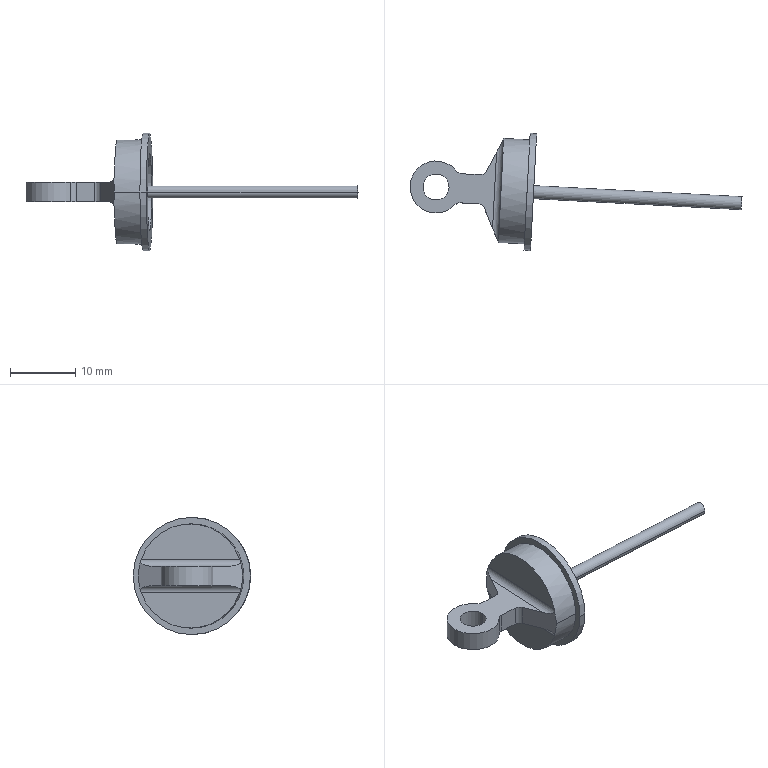Component | SolidWorks | WheelAssembly-1_DamperUpperEnd-1 | 1 solid | 29 faces | box 50.99 x 18.03 x 18 mm | volume 1080 mm3 | cylinder 17 | plane 12 | commonest cylinder face diameters 2 x8 16 x2 4 x2 18 x2 12 x2 8 x1
STEP:
#1=COLOUR_RGB('',0.7922,0.8196,0.9333);
#2=FILL_AREA_STYLE_COLOUR('',#1);
#3=FILL_AREA_STYLE('',(#2));
#4=SURFACE_STYLE_FILL_AREA(#3);
#5=SURFACE_SIDE_STYLE('',(#4));
#6=SURFACE_STYLE_USAGE(.BOTH.,#5);
#7=PRESENTATION_STYLE_ASSIGNMENT((#6));
#8=CARTESIAN_POINT('',(-12.976,-4.793,-22.066));
#9=VERTEX_POINT('',#8);
#10=CARTESIAN_POINT('',(-13.01,-5.422,-22.066));
#11=VERTEX_POINT('',#10);
#12=CARTESIAN_POINT('',(-12.993,-5.108,-22.066));
#13=DIRECTION('',(0.9986,-0.05275,-0.));
#14=DIRECTION('',(0.05275,0.9986,0.));
#15=AXIS2_PLACEMENT_3D('',#12,#13,#14);
#16=CIRCLE('',#15,0.315);
#17=EDGE_CURVE('',#9,#11,#16,.T.);
#18=ORIENTED_EDGE('',*,*,#17,.F.);
#19=CARTESIAN_POINT('',(-13.134,-4.785,-22.066));
#20=VERTEX_POINT('',#19);
#21=CARTESIAN_POINT('',(-12.819,-4.802,-22.066));
#22=DIRECTION('',(-0.9986,0.05275,0.));
#23=VECTOR('',#22,39.37);
#24=LINE('',#21,#23);
#25=EDGE_CURVE('',#9,#20,#24,.T.);
#26=ORIENTED_EDGE('',*,*,#25,.T.);
#27=CARTESIAN_POINT('',(-13.139,-4.795,-21.986));
#28=VERTEX_POINT('',#27);
#29=CARTESIAN_POINT('',(-13.139,-4.795,-21.986));
#30=CARTESIAN_POINT('',(-13.135,-4.788,-22.012));
#31=CARTESIAN_POINT('',(-13.134,-4.785,-22.039));
#32=CARTESIAN_POINT('',(-13.134,-4.785,-22.066));
#33=(BOUNDED_CURVE()B_SPLINE_CURVE(3,(#29,#30,#31,#32),.UNSPECIFIED.,.F.,.F.)B_SPLINE_CURVE_WITH_KNOTS((4,4),(6.028,6.283),.UNSPECIFIED.)CURVE()GEOMETRIC_REPRESENTATION_ITEM()RATIONAL_B_SPLINE_CURVE((1.,0.9946,0.9946,1.))REPRESENTATION_ITEM(''));
#34=EDGE_CURVE('',#28,#20,#33,.T.);
#35=ORIENTED_EDGE('',*,*,#34,.F.);
#36=CARTESIAN_POINT('',(-13.134,-4.801,-21.967));
#37=VERTEX_POINT('',#36);
#38=CARTESIAN_POINT('',(-13.139,-4.795,-21.986));
#39=CARTESIAN_POINT('',(-13.136,-4.797,-21.98));
#40=CARTESIAN_POINT('',(-13.134,-4.799,-21.974));
#41=CARTESIAN_POINT('',(-13.134,-4.801,-21.967));
#42=B_SPLINE_CURVE_WITH_KNOTS('',3,(#38,#39,#40,#41),.UNSPECIFIED.,.F.,.F.,(4,4),(0.,0.0005135),.UNSPECIFIED.);
#43=EDGE_CURVE('',#28,#37,#42,.T.);
#44=ORIENTED_EDGE('',*,*,#43,.T.);
#45=CARTESIAN_POINT('',(-13.166,-5.398,-21.967));
#46=VERTEX_POINT('',#45);
#47=CARTESIAN_POINT('',(-13.15,-5.1,-22.066));
#48=DIRECTION('',(-0.9986,0.05275,0.));
#49=DIRECTION('',(-0.05275,-0.9986,0.));
#50=AXIS2_PLACEMENT_3D('',#47,#48,#49);
#51=CIRCLE('',#50,0.315);
#52=EDGE_CURVE('',#46,#37,#51,.T.);
#53=ORIENTED_EDGE('',*,*,#52,.F.);
#54=CARTESIAN_POINT('',(-13.171,-5.404,-21.986));
#55=VERTEX_POINT('',#54);
#56=CARTESIAN_POINT('',(-13.166,-5.398,-21.967));
#57=CARTESIAN_POINT('',(-13.166,-5.4,-21.974));
#58=CARTESIAN_POINT('',(-13.168,-5.402,-21.98));
#59=CARTESIAN_POINT('',(-13.171,-5.404,-21.986));
#60=B_SPLINE_CURVE_WITH_KNOTS('',3,(#56,#57,#58,#59),.UNSPECIFIED.,.F.,.F.,(4,4),(0.,0.0005136),.UNSPECIFIED.);
#61=EDGE_CURVE('',#46,#55,#60,.T.);
#62=ORIENTED_EDGE('',*,*,#61,.T.);
#63=CARTESIAN_POINT('',(-13.167,-5.414,-22.066));
#64=VERTEX_POINT('',#63);
#65=CARTESIAN_POINT('',(-13.167,-5.414,-22.066));
#66=CARTESIAN_POINT('',(-13.167,-5.414,-22.039));
#67=CARTESIAN_POINT('',(-13.168,-5.411,-22.012));
#68=CARTESIAN_POINT('',(-13.171,-5.404,-21.986));
#69=(BOUNDED_CURVE()B_SPLINE_CURVE(3,(#65,#66,#67,#68),.UNSPECIFIED.,.F.,.F.)B_SPLINE_CURVE_WITH_KNOTS((4,4),(-0.,0.2556),.UNSPECIFIED.)CURVE()GEOMETRIC_REPRESENTATION_ITEM()RATIONAL_B_SPLINE_CURVE((1.,0.9946,0.9946,1.))REPRESENTATION_ITEM(''));
#70=EDGE_CURVE('',#64,#55,#69,.T.);
#71=ORIENTED_EDGE('',*,*,#70,.F.);
#72=CARTESIAN_POINT('',(-12.852,-5.431,-22.066));
#73=DIRECTION('',(-0.9986,0.05275,0.));
#74=VECTOR('',#73,39.37);
#75=LINE('',#72,#74);
#76=EDGE_CURVE('',#11,#64,#75,.T.);
#77=ORIENTED_EDGE('',*,*,#76,.F.);
#78=EDGE_LOOP('',(#18,#26,#35,#44,#53,#62,#71,#77));
#79=FACE_OUTER_BOUND('',#78,.T.);
#80=CARTESIAN_POINT('',(-12.836,-5.116,-22.066));
#81=DIRECTION('',(-0.9986,0.05275,0.));
#82=DIRECTION('',(-0.05275,-0.9986,0.));
#83=AXIS2_PLACEMENT_3D('',#80,#81,#82);
#84=CYLINDRICAL_SURFACE('',#83,0.315);
#85=ADVANCED_FACE('',(#79),#84,.T.);
#86=CARTESIAN_POINT('',(-13.465,-5.083,-22.007));
#87=VERTEX_POINT('',#86);
#88=CARTESIAN_POINT('',(-13.622,-5.075,-22.007));
#89=VERTEX_POINT('',#88);
#90=CARTESIAN_POINT('',(-13.543,-5.079,-22.007));
#91=DIRECTION('',(0.,0.,1.));
#92=DIRECTION('',(-0.9986,0.05275,0.));
#93=AXIS2_PLACEMENT_3D('',#90,#91,#92);
#94=CIRCLE('',#93,0.07874);
#95=EDGE_CURVE('',#87,#89,#94,.T.);
#96=ORIENTED_EDGE('',*,*,#95,.T.);
#97=CARTESIAN_POINT('',(-13.622,-5.075,-22.125));
#98=VERTEX_POINT('',#97);
#99=CARTESIAN_POINT('',(-13.622,-5.075,-22.007));
#100=DIRECTION('',(-0.,-0.,-1.));
#101=VECTOR('',#100,39.37);
#102=LINE('',#99,#101);
#103=EDGE_CURVE('',#89,#98,#102,.T.);
#104=ORIENTED_EDGE('',*,*,#103,.T.);
#105=CARTESIAN_POINT('',(-13.465,-5.083,-22.125));
#106=VERTEX_POINT('',#105);
#107=CARTESIAN_POINT('',(-13.543,-5.079,-22.125));
#108=DIRECTION('',(0.,0.,1.));
#109=DIRECTION('',(-0.9986,0.05275,0.));
#110=AXIS2_PLACEMENT_3D('',#107,#108,#109);
#111=CIRCLE('',#110,0.07874);
#112=EDGE_CURVE('',#106,#98,#111,.T.);
#113=ORIENTED_EDGE('',*,*,#112,.F.);
#114=CARTESIAN_POINT('',(-13.465,-5.083,-22.007));
#115=DIRECTION('',(-0.,-0.,-1.));
#116=VECTOR('',#115,39.37);
#117=LINE('',#114,#116);
#118=EDGE_CURVE('',#87,#106,#117,.T.);
#119=ORIENTED_EDGE('',*,*,#118,.F.);
#120=EDGE_LOOP('',(#96,#104,#113,#119));
#121=FACE_OUTER_BOUND('',#120,.T.);
#122=CARTESIAN_POINT('',(-13.543,-5.079,-22.007));
#123=DIRECTION('',(-0.,-0.,-1.));
#124=DIRECTION('',(0.9986,-0.05275,0.));
#125=AXIS2_PLACEMENT_3D('',#122,#123,#124);
#126=CYLINDRICAL_SURFACE('',#125,0.07874);
#127=ADVANCED_FACE('',(#121),#126,.F.);
#128=CARTESIAN_POINT('',(-12.974,-4.754,-22.066));
#129=VERTEX_POINT('',#128);
#130=CARTESIAN_POINT('',(-13.012,-5.462,-22.066));
#131=VERTEX_POINT('',#130);
#132=CARTESIAN_POINT('',(-12.993,-5.108,-22.066));
#133=DIRECTION('',(0.9986,-0.05275,-0.));
#134=DIRECTION('',(0.05275,0.9986,0.));
#135=AXIS2_PLACEMENT_3D('',#132,#133,#134);
#136=CIRCLE('',#135,0.3543);
#137=EDGE_CURVE('',#129,#131,#136,.T.);
#138=ORIENTED_EDGE('',*,*,#137,.T.);
#139=CARTESIAN_POINT('',(-12.972,-5.464,-22.066));
#140=VERTEX_POINT('',#139);
#141=CARTESIAN_POINT('',(-13.012,-5.462,-22.066));
#142=DIRECTION('',(0.9986,-0.05275,-0.));
#143=VECTOR('',#142,39.37);
#144=LINE('',#141,#143);
#145=EDGE_CURVE('',#131,#140,#144,.T.);
#146=ORIENTED_EDGE('',*,*,#145,.T.);
#147=CARTESIAN_POINT('',(-12.935,-4.756,-22.066));
#148=VERTEX_POINT('',#147);
#149=CARTESIAN_POINT('',(-12.954,-5.11,-22.066));
#150=DIRECTION('',(0.9986,-0.05275,-0.));
#151=DIRECTION('',(0.05275,0.9986,0.));
#152=AXIS2_PLACEMENT_3D('',#149,#150,#151);
#153=CIRCLE('',#152,0.3543);
#154=EDGE_CURVE('',#148,#140,#153,.T.);
#155=ORIENTED_EDGE('',*,*,#154,.F.);
#156=CARTESIAN_POINT('',(-12.974,-4.754,-22.066));
#157=DIRECTION('',(0.9986,-0.05275,-0.));
#158=VECTOR('',#157,39.37);
#159=LINE('',#156,#158);
#160=EDGE_CURVE('',#129,#148,#159,.T.);
#161=ORIENTED_EDGE('',*,*,#160,.F.);
#162=EDGE_LOOP('',(#138,#146,#155,#161));
#163=FACE_OUTER_BOUND('',#162,.T.);
#164=CARTESIAN_POINT('',(-12.993,-5.108,-22.066));
#165=DIRECTION('',(0.9986,-0.05275,-0.));
#166=DIRECTION('',(0.05275,0.9986,0.));
#167=AXIS2_PLACEMENT_3D('',#164,#165,#166);
#168=CYLINDRICAL_SURFACE('',#167,0.3543);
#169=ADVANCED_FACE('',(#163),#168,.T.);
#170=CARTESIAN_POINT('',(-11.693,-5.137,-22.066));
#171=VERTEX_POINT('',#170);
#172=CARTESIAN_POINT('',(-11.698,-5.216,-22.066));
#173=VERTEX_POINT('',#172);
#174=CARTESIAN_POINT('',(-11.695,-5.176,-22.066));
#175=DIRECTION('',(0.9986,-0.05275,-0.));
#176=DIRECTION('',(0.05275,0.9986,0.));
#177=AXIS2_PLACEMENT_3D('',#174,#175,#176);
#178=CIRCLE('',#177,0.03937);
#179=EDGE_CURVE('',#171,#173,#178,.T.);
#180=ORIENTED_EDGE('',*,*,#179,.F.);
#181=CARTESIAN_POINT('',(-13.069,-5.064,-22.066));
#182=VERTEX_POINT('',#181);
#183=CARTESIAN_POINT('',(-11.693,-5.137,-22.066));
#184=DIRECTION('',(-0.9986,0.05275,0.));
#185=VECTOR('',#184,39.37);
#186=LINE('',#183,#185);
#187=EDGE_CURVE('',#171,#182,#186,.T.);
#188=ORIENTED_EDGE('',*,*,#187,.T.);
#189=CARTESIAN_POINT('',(-13.074,-5.143,-22.066));
#190=VERTEX_POINT('',#189);
#191=CARTESIAN_POINT('',(-13.072,-5.104,-22.066));
#192=DIRECTION('',(0.9986,-0.05275,-0.));
#193=DIRECTION('',(-0.05275,-0.9986,0.));
#194=AXIS2_PLACEMENT_3D('',#191,#192,#193);
#195=CIRCLE('',#194,0.03937);
#196=EDGE_CURVE('',#182,#190,#195,.T.);
#197=ORIENTED_EDGE('',*,*,#196,.T.);
#198=CARTESIAN_POINT('',(-11.698,-5.216,-22.066));
#199=DIRECTION('',(-0.9986,0.05275,0.));
#200=VECTOR('',#199,39.37);
#201=LINE('',#198,#200);
#202=EDGE_CURVE('',#173,#190,#201,.T.);
#203=ORIENTED_EDGE('',*,*,#202,.F.);
#204=EDGE_LOOP('',(#180,#188,#197,#203));
#205=FACE_OUTER_BOUND('',#204,.T.);
#206=CARTESIAN_POINT('',(-11.695,-5.176,-22.066));
#207=DIRECTION('',(-0.9986,0.05275,0.));
#208=DIRECTION('',(-0.05275,-0.9986,0.));
#209=AXIS2_PLACEMENT_3D('',#206,#207,#208);
#210=CYLINDRICAL_SURFACE('',#209,0.03937);
#211=ADVANCED_FACE('',(#205),#210,.T.);
#212=CARTESIAN_POINT('',(-12.941,-4.874,-22.066));
#213=VERTEX_POINT('',#212);
#214=CARTESIAN_POINT('',(-12.966,-5.346,-22.066));
#215=VERTEX_POINT('',#214);
#216=CARTESIAN_POINT('',(-12.954,-5.11,-22.066));
#217=DIRECTION('',(-0.9986,0.05275,0.));
#218=DIRECTION('',(-0.05275,-0.9986,0.));
#219=AXIS2_PLACEMENT_3D('',#216,#217,#218);
#220=CIRCLE('',#219,0.2362);
#221=EDGE_CURVE('',#213,#215,#220,.T.);
#222=ORIENTED_EDGE('',*,*,#221,.F.);
#223=CARTESIAN_POINT('',(-13.059,-4.868,-22.066));
#224=VERTEX_POINT('',#223);
#225=CARTESIAN_POINT('',(-12.823,-4.88,-22.066));
#226=DIRECTION('',(-0.9986,0.05275,0.));
#227=VECTOR('',#226,39.37);
#228=LINE('',#225,#227);
#229=EDGE_CURVE('',#213,#224,#228,.T.);
#230=ORIENTED_EDGE('',*,*,#229,.T.);
#231=CARTESIAN_POINT('',(-13.084,-5.34,-22.066));
#232=VERTEX_POINT('',#231);
#233=CARTESIAN_POINT('',(-13.072,-5.104,-22.066));
#234=DIRECTION('',(-0.9986,0.05275,0.));
#235=DIRECTION('',(-0.05275,-0.9986,0.));
#236=AXIS2_PLACEMENT_3D('',#233,#234,#235);
#237=CIRCLE('',#236,0.2362);
#238=EDGE_CURVE('',#224,#232,#237,.T.);
#239=ORIENTED_EDGE('',*,*,#238,.T.);
#240=CARTESIAN_POINT('',(-12.848,-5.352,-22.066));
#241=DIRECTION('',(-0.9986,0.05275,0.));
#242=VECTOR('',#241,39.37);
#243=LINE('',#240,#242);
#244=EDGE_CURVE('',#215,#232,#243,.T.);
#245=ORIENTED_EDGE('',*,*,#244,.F.);
#246=EDGE_LOOP('',(#222,#230,#239,#245));
#247=FACE_OUTER_BOUND('',#246,.T.);
#248=CARTESIAN_POINT('',(-12.836,-5.116,-22.066));
#249=DIRECTION('',(-0.9986,0.05275,0.));
#250=DIRECTION('',(-0.05275,-0.9986,0.));
#251=AXIS2_PLACEMENT_3D('',#248,#249,#250);
#252=CYLINDRICAL_SURFACE('',#251,0.2362);
#253=ADVANCED_FACE('',(#247),#252,.F.);
#254=CARTESIAN_POINT('',(-12.954,-5.11,-22.066));
#255=DIRECTION('',(-0.9986,0.05275,0.));
#256=DIRECTION('',(-0.05275,-0.9986,0.));
#257=AXIS2_PLACEMENT_3D('',#254,#255,#256);
#258=CIRCLE('',#257,0.2362);
#259=EDGE_CURVE('',#215,#213,#258,.T.);
#260=ORIENTED_EDGE('',*,*,#259,.T.);
#261=ORIENTED_EDGE('',*,*,#221,.T.);
#262=EDGE_LOOP('',(#260,#261));
#263=FACE_BOUND('',#262,.T.);
#264=ORIENTED_EDGE('',*,*,#154,.T.);
#265=CARTESIAN_POINT('',(-12.954,-5.11,-22.066));
#266=DIRECTION('',(0.9986,-0.05275,-0.));
#267=DIRECTION('',(0.05275,0.9986,0.));
#268=AXIS2_PLACEMENT_3D('',#265,#266,#267);
#269=CIRCLE('',#268,0.3543);
#270=EDGE_CURVE('',#140,#148,#269,.T.);
#271=ORIENTED_EDGE('',*,*,#270,.T.);
#272=EDGE_LOOP('',(#264,#271));
#273=FACE_OUTER_BOUND('',#272,.T.);
#274=CARTESIAN_POINT('',(-12.954,-5.11,-22.066));
#275=DIRECTION('',(-0.9986,0.05275,0.));
#276=DIRECTION('',(-0.05275,-0.9986,0.));
#277=AXIS2_PLACEMENT_3D('',#274,#275,#276);
#278=PLANE('',#277);
#279=ADVANCED_FACE('',(#263,#273),#278,.F.);
#280=ORIENTED_EDGE('',*,*,#229,.F.);
#281=ORIENTED_EDGE('',*,*,#259,.F.);
#282=ORIENTED_EDGE('',*,*,#244,.T.);
#283=CARTESIAN_POINT('',(-13.072,-5.104,-22.066));
#284=DIRECTION('',(-0.9986,0.05275,0.));
#285=DIRECTION('',(-0.05275,-0.9986,0.));
#286=AXIS2_PLACEMENT_3D('',#283,#284,#285);
#287=CIRCLE('',#286,0.2362);
#288=EDGE_CURVE('',#232,#224,#287,.T.);
#289=ORIENTED_EDGE('',*,*,#288,.T.);
#290=EDGE_LOOP('',(#280,#281,#282,#289));
#291=FACE_OUTER_BOUND('',#290,.T.);
#292=CARTESIAN_POINT('',(-12.836,-5.116,-22.066));
#293=DIRECTION('',(-0.9986,0.05275,0.));
#294=DIRECTION('',(-0.05275,-0.9986,0.));
#295=AXIS2_PLACEMENT_3D('',#292,#293,#294);
#296=CYLINDRICAL_SURFACE('',#295,0.2362);
#297=ADVANCED_FACE('',(#291),#296,.F.);
#298=CARTESIAN_POINT('',(-13.072,-5.104,-22.066));
#299=DIRECTION('',(0.9986,-0.05275,-0.));
#300=DIRECTION('',(-0.05275,-0.9986,0.));
#301=AXIS2_PLACEMENT_3D('',#298,#299,#300);
#302=CIRCLE('',#301,0.03937);
#303=EDGE_CURVE('',#190,#182,#302,.T.);
#304=ORIENTED_EDGE('',*,*,#303,.F.);
#305=ORIENTED_EDGE('',*,*,#196,.F.);
#306=EDGE_LOOP('',(#304,#305));
#307=FACE_BOUND('',#306,.T.);
#308=ORIENTED_EDGE('',*,*,#288,.F.);
#309=ORIENTED_EDGE('',*,*,#238,.F.);
#310=EDGE_LOOP('',(#308,#309));
#311=FACE_OUTER_BOUND('',#310,.T.);
#312=CARTESIAN_POINT('',(-13.072,-5.104,-22.066));
#313=DIRECTION('',(-0.9986,0.05275,0.));
#314=DIRECTION('',(-0.05275,-0.9986,0.));
#315=AXIS2_PLACEMENT_3D('',#312,#313,#314);
#316=PLANE('',#315);
#317=ADVANCED_FACE('',(#307,#311),#316,.F.);
#318=ORIENTED_EDGE('',*,*,#187,.F.);
#319=CARTESIAN_POINT('',(-11.695,-5.176,-22.066));
#320=DIRECTION('',(0.9986,-0.05275,-0.));
#321=DIRECTION('',(0.05275,0.9986,0.));
#322=AXIS2_PLACEMENT_3D('',#319,#320,#321);
#323=CIRCLE('',#322,0.03937);
#324=EDGE_CURVE('',#173,#171,#323,.T.);
#325=ORIENTED_EDGE('',*,*,#324,.F.);
#326=ORIENTED_EDGE('',*,*,#202,.T.);
#327=ORIENTED_EDGE('',*,*,#303,.T.);
#328=EDGE_LOOP('',(#318,#325,#326,#327));
#329=FACE_OUTER_BOUND('',#328,.T.);
#330=CARTESIAN_POINT('',(-11.695,-5.176,-22.066));
#331=DIRECTION('',(-0.9986,0.05275,0.));
#332=DIRECTION('',(-0.05275,-0.9986,0.));
#333=AXIS2_PLACEMENT_3D('',#330,#331,#332);
#334=CYLINDRICAL_SURFACE('',#333,0.03937);
#335=ADVANCED_FACE('',(#329),#334,.T.);
#336=ORIENTED_EDGE('',*,*,#324,.T.);
#337=ORIENTED_EDGE('',*,*,#179,.T.);
#338=EDGE_LOOP('',(#336,#337));
#339=FACE_OUTER_BOUND('',#338,.T.);
#340=CARTESIAN_POINT('',(-11.695,-5.176,-22.066));
#341=DIRECTION('',(0.9986,-0.05275,-0.));
#342=DIRECTION('',(0.05275,0.9986,-0.));
#343=AXIS2_PLACEMENT_3D('',#340,#341,#342);
#344=PLANE('',#343);
#345=ADVANCED_FACE('',(#339),#344,.T.);
#346=ORIENTED_EDGE('',*,*,#145,.F.);
#347=CARTESIAN_POINT('',(-12.993,-5.108,-22.066));
#348=DIRECTION('',(0.9986,-0.05275,-0.));
#349=DIRECTION('',(0.05275,0.9986,0.));
#350=AXIS2_PLACEMENT_3D('',#347,#348,#349);
#351=CIRCLE('',#350,0.3543);
#352=EDGE_CURVE('',#131,#129,#351,.T.);
#353=ORIENTED_EDGE('',*,*,#352,.T.);
#354=ORIENTED_EDGE('',*,*,#160,.T.);
#355=ORIENTED_EDGE('',*,*,#270,.F.);
#356=EDGE_LOOP('',(#346,#353,#354,#355));
#357=FACE_OUTER_BOUND('',#356,.T.);
#358=CARTESIAN_POINT('',(-12.993,-5.108,-22.066));
#359=DIRECTION('',(0.9986,-0.05275,-0.));
#360=DIRECTION('',(0.05275,0.9986,0.));
#361=AXIS2_PLACEMENT_3D('',#358,#359,#360);
#362=CYLINDRICAL_SURFACE('',#361,0.3543);
#363=ADVANCED_FACE('',(#357),#362,.T.);
#364=CARTESIAN_POINT('',(-12.993,-5.108,-22.066));
#365=DIRECTION('',(0.9986,-0.05275,-0.));
#366=DIRECTION('',(0.05275,0.9986,0.));
#367=AXIS2_PLACEMENT_3D('',#364,#365,#366);
#368=CIRCLE('',#367,0.315);
#369=EDGE_CURVE('',#11,#9,#368,.T.);
#370=ORIENTED_EDGE('',*,*,#369,.T.);
#371=ORIENTED_EDGE('',*,*,#17,.T.);
#372=EDGE_LOOP('',(#370,#371));
#373=FACE_BOUND('',#372,.T.);
#374=ORIENTED_EDGE('',*,*,#137,.F.);
#375=ORIENTED_EDGE('',*,*,#352,.F.);
#376=EDGE_LOOP('',(#374,#375));
#377=FACE_OUTER_BOUND('',#376,.T.);
#378=CARTESIAN_POINT('',(-12.993,-5.108,-22.066));
#379=DIRECTION('',(0.9986,-0.05275,-0.));
#380=DIRECTION('',(0.05275,0.9986,-0.));
#381=AXIS2_PLACEMENT_3D('',#378,#379,#380);
#382=PLANE('',#381);
#383=ADVANCED_FACE('',(#373,#377),#382,.F.);
#384=ORIENTED_EDGE('',*,*,#103,.F.);
#385=CARTESIAN_POINT('',(-13.543,-5.079,-22.007));
#386=DIRECTION('',(0.,0.,1.));
#387=DIRECTION('',(-0.9986,0.05275,0.));
#388=AXIS2_PLACEMENT_3D('',#385,#386,#387);
#389=CIRCLE('',#388,0.07874);
#390=EDGE_CURVE('',#89,#87,#389,.T.);
#391=ORIENTED_EDGE('',*,*,#390,.T.);
#392=ORIENTED_EDGE('',*,*,#118,.T.);
#393=CARTESIAN_POINT('',(-13.543,-5.079,-22.125));
#394=DIRECTION('',(0.,0.,1.));
#395=DIRECTION('',(-0.9986,0.05275,0.));
#396=AXIS2_PLACEMENT_3D('',#393,#394,#395);
#397=CIRCLE('',#396,0.07874);
#398=EDGE_CURVE('',#98,#106,#397,.T.);
#399=ORIENTED_EDGE('',*,*,#398,.F.);
#400=EDGE_LOOP('',(#384,#391,#392,#399));
#401=FACE_OUTER_BOUND('',#400,.T.);
#402=CARTESIAN_POINT('',(-13.543,-5.079,-22.007));
#403=DIRECTION('',(-0.,-0.,-1.));
#404=DIRECTION('',(0.9986,-0.05275,0.));
#405=AXIS2_PLACEMENT_3D('',#402,#403,#404);
#406=CYLINDRICAL_SURFACE('',#405,0.07874);
#407=ADVANCED_FACE('',(#401),#406,.F.);
#408=CARTESIAN_POINT('',(-13.398,-5.175,-22.007));
#409=VERTEX_POINT('',#408);
#410=CARTESIAN_POINT('',(-13.285,-5.181,-22.007));
#411=VERTEX_POINT('',#410);
#412=CARTESIAN_POINT('',(-13.26,-5.182,-22.007));
#413=DIRECTION('',(0.9986,-0.05275,-0.));
#414=VECTOR('',#413,39.37);
#415=LINE('',#412,#414);
#416=EDGE_CURVE('',#409,#411,#415,.T.);
#417=ORIENTED_EDGE('',*,*,#416,.F.);
#418=CARTESIAN_POINT('',(-13.398,-5.175,-22.125));
#419=VERTEX_POINT('',#418);
#420=CARTESIAN_POINT('',(-13.398,-5.175,-22.125));
#421=DIRECTION('',(-0.,-0.,-1.));
#422=VECTOR('',#421,39.37);
#423=LINE('',#420,#422);
#424=EDGE_CURVE('',#409,#419,#423,.T.);
#425=ORIENTED_EDGE('',*,*,#424,.T.);
#426=CARTESIAN_POINT('',(-13.285,-5.181,-22.125));
#427=VERTEX_POINT('',#426);
#428=CARTESIAN_POINT('',(-13.26,-5.182,-22.125));
#429=DIRECTION('',(0.9986,-0.05275,-0.));
#430=VECTOR('',#429,39.37);
#431=LINE('',#428,#430);
#432=EDGE_CURVE('',#419,#427,#431,.T.);
#433=ORIENTED_EDGE('',*,*,#432,.T.);
#434=CARTESIAN_POINT('',(-13.285,-5.181,-22.007));
#435=DIRECTION('',(0.,0.,1.));
#436=VECTOR('',#435,39.37);
#437=LINE('',#434,#436);
#438=EDGE_CURVE('',#427,#411,#437,.T.);
#439=ORIENTED_EDGE('',*,*,#438,.T.);
#440=EDGE_LOOP('',(#417,#425,#433,#439));
#441=FACE_OUTER_BOUND('',#440,.T.);
#442=CARTESIAN_POINT('',(-13.26,-5.182,-22.007));
#443=DIRECTION('',(0.05275,0.9986,-0.));
#444=DIRECTION('',(-0.9986,0.05275,0.));
#445=AXIS2_PLACEMENT_3D('',#442,#443,#444);
#446=PLANE('',#445);
#447=ADVANCED_FACE('',(#441),#446,.F.);
#448=CARTESIAN_POINT('',(-13.429,-5.187,-22.007));
#449=VERTEX_POINT('',#448);
#450=CARTESIAN_POINT('',(-13.4,-5.214,-22.007));
#451=DIRECTION('',(-0.,-0.,-1.));
#452=DIRECTION('',(-0.9986,0.05275,0.));
#453=AXIS2_PLACEMENT_3D('',#450,#451,#452);
#454=CIRCLE('',#453,0.03937);
#455=EDGE_CURVE('',#449,#409,#454,.T.);
#456=ORIENTED_EDGE('',*,*,#455,.F.);
#457=CARTESIAN_POINT('',(-13.429,-5.187,-22.125));
#458=VERTEX_POINT('',#457);
#459=CARTESIAN_POINT('',(-13.429,-5.187,-22.007));
#460=DIRECTION('',(0.,0.,1.));
#461=VECTOR('',#460,39.37);
#462=LINE('',#459,#461);
#463=EDGE_CURVE('',#458,#449,#462,.T.);
#464=ORIENTED_EDGE('',*,*,#463,.F.);
#465=CARTESIAN_POINT('',(-13.4,-5.214,-22.125));
#466=DIRECTION('',(0.,0.,1.));
#467=DIRECTION('',(-0.9986,0.05275,0.));
#468=AXIS2_PLACEMENT_3D('',#465,#466,#467);
#469=CIRCLE('',#468,0.03937);
#470=EDGE_CURVE('',#419,#458,#469,.T.);
#471=ORIENTED_EDGE('',*,*,#470,.F.);
#472=ORIENTED_EDGE('',*,*,#424,.F.);
#473=EDGE_LOOP('',(#456,#464,#471,#472));
#474=FACE_OUTER_BOUND('',#473,.T.);
#475=CARTESIAN_POINT('',(-13.4,-5.214,-22.007));
#476=DIRECTION('',(-0.,-0.,-1.));
#477=DIRECTION('',(0.9986,-0.05275,0.));
#478=AXIS2_PLACEMENT_3D('',#475,#476,#477);
#479=CYLINDRICAL_SURFACE('',#478,0.03937);
#480=ADVANCED_FACE('',(#474),#479,.F.);
#481=CARTESIAN_POINT('',(-13.418,-4.983,-22.007));
#482=VERTEX_POINT('',#481);
#483=CARTESIAN_POINT('',(-13.543,-5.079,-22.007));
#484=DIRECTION('',(0.,0.,1.));
#485=DIRECTION('',(-0.9986,0.05275,0.));
#486=AXIS2_PLACEMENT_3D('',#483,#484,#485);
#487=CIRCLE('',#486,0.1575);
#488=EDGE_CURVE('',#482,#449,#487,.T.);
#489=ORIENTED_EDGE('',*,*,#488,.F.);
#490=CARTESIAN_POINT('',(-13.418,-4.983,-22.125));
#491=VERTEX_POINT('',#490);
#492=CARTESIAN_POINT('',(-13.418,-4.983,-22.007));
#493=DIRECTION('',(-0.,-0.,-1.));
#494=VECTOR('',#493,39.37);
#495=LINE('',#492,#494);
#496=EDGE_CURVE('',#482,#491,#495,.T.);
#497=ORIENTED_EDGE('',*,*,#496,.T.);
#498=CARTESIAN_POINT('',(-13.543,-5.079,-22.125));
#499=DIRECTION('',(0.,0.,1.));
#500=DIRECTION('',(-0.9986,0.05275,0.));
#501=AXIS2_PLACEMENT_3D('',#498,#499,#500);
#502=CIRCLE('',#501,0.1575);
#503=EDGE_CURVE('',#491,#458,#502,.T.);
#504=ORIENTED_EDGE('',*,*,#503,.T.);
#505=ORIENTED_EDGE('',*,*,#463,.T.);
#506=EDGE_LOOP('',(#489,#497,#504,#505));
#507=FACE_OUTER_BOUND('',#506,.T.);
#508=CARTESIAN_POINT('',(-13.543,-5.079,-22.007));
#509=DIRECTION('',(-0.,-0.,-1.));
#510=DIRECTION('',(0.9986,-0.05275,0.));
#511=AXIS2_PLACEMENT_3D('',#508,#509,#510);
#512=CYLINDRICAL_SURFACE('',#511,0.1575);
#513=ADVANCED_FACE('',(#507),#512,.T.);
#514=CARTESIAN_POINT('',(-13.389,-4.999,-22.007));
#515=VERTEX_POINT('',#514);
#516=CARTESIAN_POINT('',(-13.387,-4.959,-22.007));
#517=DIRECTION('',(-0.,-0.,-1.));
#518=DIRECTION('',(-0.9986,0.05275,0.));
#519=AXIS2_PLACEMENT_3D('',#516,#517,#518);
#520=CIRCLE('',#519,0.03937);
#521=EDGE_CURVE('',#515,#482,#520,.T.);
#522=ORIENTED_EDGE('',*,*,#521,.F.);
#523=CARTESIAN_POINT('',(-13.389,-4.999,-22.125));
#524=VERTEX_POINT('',#523);
#525=CARTESIAN_POINT('',(-13.389,-4.999,-22.007));
#526=DIRECTION('',(0.,0.,1.));
#527=VECTOR('',#526,39.37);
#528=LINE('',#525,#527);
#529=EDGE_CURVE('',#524,#515,#528,.T.);
#530=ORIENTED_EDGE('',*,*,#529,.F.);
#531=CARTESIAN_POINT('',(-13.387,-4.959,-22.125));
#532=DIRECTION('',(0.,0.,1.));
#533=DIRECTION('',(-0.9986,0.05275,0.));
#534=AXIS2_PLACEMENT_3D('',#531,#532,#533);
#535=CIRCLE('',#534,0.03937);
#536=EDGE_CURVE('',#491,#524,#535,.T.);
#537=ORIENTED_EDGE('',*,*,#536,.F.);
#538=ORIENTED_EDGE('',*,*,#496,.F.);
#539=EDGE_LOOP('',(#522,#530,#537,#538));
#540=FACE_OUTER_BOUND('',#539,.T.);
#541=CARTESIAN_POINT('',(-13.387,-4.959,-22.007));
#542=DIRECTION('',(-0.,-0.,-1.));
#543=DIRECTION('',(0.9986,-0.05275,0.));
#544=AXIS2_PLACEMENT_3D('',#541,#542,#543);
#545=CYLINDRICAL_SURFACE('',#544,0.03937);
#546=ADVANCED_FACE('',(#540),#545,.F.);
#547=CARTESIAN_POINT('',(-13.276,-5.005,-22.007));
#548=VERTEX_POINT('',#547);
#549=CARTESIAN_POINT('',(-13.251,-5.006,-22.007));
#550=DIRECTION('',(-0.9986,0.05275,0.));
#551=VECTOR('',#550,39.37);
#552=LINE('',#549,#551);
#553=EDGE_CURVE('',#548,#515,#552,.T.);
#554=ORIENTED_EDGE('',*,*,#553,.F.);
#555=CARTESIAN_POINT('',(-13.276,-5.005,-22.125));
#556=VERTEX_POINT('',#555);
#557=CARTESIAN_POINT('',(-13.276,-5.005,-22.125));
#558=DIRECTION('',(-0.,-0.,-1.));
#559=VECTOR('',#558,39.37);
#560=LINE('',#557,#559);
#561=EDGE_CURVE('',#548,#556,#560,.T.);
#562=ORIENTED_EDGE('',*,*,#561,.T.);
#563=CARTESIAN_POINT('',(-13.251,-5.006,-22.125));
#564=DIRECTION('',(-0.9986,0.05275,0.));
#565=VECTOR('',#564,39.37);
#566=LINE('',#563,#565);
#567=EDGE_CURVE('',#556,#524,#566,.T.);
#568=ORIENTED_EDGE('',*,*,#567,.T.);
#569=ORIENTED_EDGE('',*,*,#529,.T.);
#570=EDGE_LOOP('',(#554,#562,#568,#569));
#571=FACE_OUTER_BOUND('',#570,.T.);
#572=CARTESIAN_POINT('',(-13.251,-5.006,-22.007));
#573=DIRECTION('',(-0.05275,-0.9986,0.));
#574=DIRECTION('',(0.9986,-0.05275,-0.));
#575=AXIS2_PLACEMENT_3D('',#572,#573,#574);
#576=PLANE('',#575);
#577=ADVANCED_FACE('',(#571),#576,.F.);
#578=CARTESIAN_POINT('',(-13.239,-4.984,-22.007));
#579=VERTEX_POINT('',#578);
#580=CARTESIAN_POINT('',(-13.274,-4.965,-22.007));
#581=DIRECTION('',(-0.,-0.,-1.));
#582=DIRECTION('',(-0.9986,0.05275,0.));
#583=AXIS2_PLACEMENT_3D('',#580,#581,#582);
#584=CIRCLE('',#583,0.03937);
#585=EDGE_CURVE('',#579,#548,#584,.T.);
#586=ORIENTED_EDGE('',*,*,#585,.F.);
#587=CARTESIAN_POINT('',(-13.239,-4.984,-22.125));
#588=VERTEX_POINT('',#587);
#589=CARTESIAN_POINT('',(-13.239,-4.984,-22.007));
#590=DIRECTION('',(0.,0.,1.));
#591=VECTOR('',#590,39.37);
#592=LINE('',#589,#591);
#593=EDGE_CURVE('',#588,#579,#592,.T.);
#594=ORIENTED_EDGE('',*,*,#593,.F.);
#595=CARTESIAN_POINT('',(-13.274,-4.965,-22.125));
#596=DIRECTION('',(0.,0.,1.));
#597=DIRECTION('',(-0.9986,0.05275,0.));
#598=AXIS2_PLACEMENT_3D('',#595,#596,#597);
#599=CIRCLE('',#598,0.03937);
#600=EDGE_CURVE('',#556,#588,#599,.T.);
#601=ORIENTED_EDGE('',*,*,#600,.F.);
#602=ORIENTED_EDGE('',*,*,#561,.F.);
#603=EDGE_LOOP('',(#586,#594,#601,#602));
#604=FACE_OUTER_BOUND('',#603,.T.);
#605=CARTESIAN_POINT('',(-13.274,-4.965,-22.007));
#606=DIRECTION('',(0.,0.,1.));
#607=DIRECTION('',(-0.9986,0.05275,0.));
#608=AXIS2_PLACEMENT_3D('',#605,#606,#607);
#609=CYLINDRICAL_SURFACE('',#608,0.03937);
#610=ADVANCED_FACE('',(#604),#609,.F.);
#611=CARTESIAN_POINT('',(-13.177,-4.867,-22.125));
#612=VERTEX_POINT('',#611);
#613=CARTESIAN_POINT('',(-13.134,-4.785,-22.125));
#614=DIRECTION('',(-0.4698,-0.8828,0.));
#615=VECTOR('',#614,39.37);
#616=LINE('',#613,#615);
#617=EDGE_CURVE('',#612,#588,#616,.T.);
#618=ORIENTED_EDGE('',*,*,#617,.F.);
#619=CARTESIAN_POINT('',(-13.202,-5.328,-22.125));
#620=VERTEX_POINT('',#619);
#621=CARTESIAN_POINT('',(-13.189,-5.097,-22.125));
#622=DIRECTION('',(-0.05275,-0.9986,0.));
#623=VECTOR('',#622,39.37);
#624=LINE('',#621,#623);
#625=EDGE_CURVE('',#612,#620,#624,.T.);
#626=ORIENTED_EDGE('',*,*,#625,.T.);
#627=CARTESIAN_POINT('',(-13.251,-5.205,-22.125));
#628=VERTEX_POINT('',#627);
#629=CARTESIAN_POINT('',(-13.167,-5.414,-22.125));
#630=DIRECTION('',(0.3742,-0.9273,0.));
#631=VECTOR('',#630,39.37);
#632=LINE('',#629,#631);
#633=EDGE_CURVE('',#628,#620,#632,.T.);
#634=ORIENTED_EDGE('',*,*,#633,.F.);
#635=CARTESIAN_POINT('',(-13.288,-5.22,-22.125));
#636=DIRECTION('',(0.,0.,1.));
#637=DIRECTION('',(-0.9986,0.05275,0.));
#638=AXIS2_PLACEMENT_3D('',#635,#636,#637);
#639=CIRCLE('',#638,0.03937);
#640=EDGE_CURVE('',#628,#427,#639,.T.);
#641=ORIENTED_EDGE('',*,*,#640,.T.);
#642=ORIENTED_EDGE('',*,*,#432,.F.);
#643=ORIENTED_EDGE('',*,*,#470,.T.);
#644=ORIENTED_EDGE('',*,*,#503,.F.);
#645=ORIENTED_EDGE('',*,*,#536,.T.);
#646=ORIENTED_EDGE('',*,*,#567,.F.);
#647=ORIENTED_EDGE('',*,*,#600,.T.);
#648=EDGE_LOOP('',(#618,#626,#634,#641,#642,#643,#644,#645,#646,#647));
#649=FACE_OUTER_BOUND('',#648,.T.);
#650=ORIENTED_EDGE('',*,*,#112,.T.);
#651=ORIENTED_EDGE('',*,*,#398,.T.);
#652=EDGE_LOOP('',(#650,#651));
#653=FACE_BOUND('',#652,.T.);
#654=CARTESIAN_POINT('',(-13.543,-5.079,-22.125));
#655=DIRECTION('',(0.,0.,1.));
#656=DIRECTION('',(-0.9986,0.05275,0.));
#657=AXIS2_PLACEMENT_3D('',#654,#655,#656);
#658=PLANE('',#657);
#659=ADVANCED_FACE('',(#649,#653),#658,.F.);
#660=CARTESIAN_POINT('',(-13.251,-5.205,-22.007));
#661=VERTEX_POINT('',#660);
#662=CARTESIAN_POINT('',(-13.288,-5.22,-22.007));
#663=DIRECTION('',(-0.,-0.,-1.));
#664=DIRECTION('',(-0.9986,0.05275,0.));
#665=AXIS2_PLACEMENT_3D('',#662,#663,#664);
#666=CIRCLE('',#665,0.03937);
#667=EDGE_CURVE('',#411,#661,#666,.T.);
#668=ORIENTED_EDGE('',*,*,#667,.F.);
#669=ORIENTED_EDGE('',*,*,#438,.F.);
#670=ORIENTED_EDGE('',*,*,#640,.F.);
#671=CARTESIAN_POINT('',(-13.251,-5.205,-22.125));
#672=DIRECTION('',(-0.,-0.,-1.));
#673=VECTOR('',#672,39.37);
#674=LINE('',#671,#673);
#675=EDGE_CURVE('',#661,#628,#674,.T.);
#676=ORIENTED_EDGE('',*,*,#675,.F.);
#677=EDGE_LOOP('',(#668,#669,#670,#676));
#678=FACE_OUTER_BOUND('',#677,.T.);
#679=CARTESIAN_POINT('',(-13.288,-5.22,-22.007));
#680=DIRECTION('',(0.,0.,1.));
#681=DIRECTION('',(-0.9986,0.05275,0.));
#682=AXIS2_PLACEMENT_3D('',#679,#680,#681);
#683=CYLINDRICAL_SURFACE('',#682,0.03937);
#684=ADVANCED_FACE('',(#678),#683,.F.);
#685=CARTESIAN_POINT('',(-13.202,-5.328,-22.007));
#686=VERTEX_POINT('',#685);
#687=CARTESIAN_POINT('',(-13.167,-5.414,-22.007));
#688=DIRECTION('',(0.3742,-0.9273,0.));
#689=VECTOR('',#688,39.37);
#690=LINE('',#687,#689);
#691=EDGE_CURVE('',#661,#686,#690,.T.);
#692=ORIENTED_EDGE('',*,*,#691,.T.);
#693=CARTESIAN_POINT('',(-13.177,-4.867,-22.007));
#694=VERTEX_POINT('',#693);
#695=CARTESIAN_POINT('',(-13.173,-4.788,-22.007));
#696=DIRECTION('',(0.05275,0.9986,-0.));
#697=VECTOR('',#696,39.37);
#698=LINE('',#695,#697);
#699=EDGE_CURVE('',#686,#694,#698,.T.);
#700=ORIENTED_EDGE('',*,*,#699,.T.);
#701=CARTESIAN_POINT('',(-13.134,-4.785,-22.007));
#702=DIRECTION('',(-0.4698,-0.8828,0.));
#703=VECTOR('',#702,39.37);
#704=LINE('',#701,#703);
#705=EDGE_CURVE('',#694,#579,#704,.T.);
#706=ORIENTED_EDGE('',*,*,#705,.T.);
#707=ORIENTED_EDGE('',*,*,#585,.T.);
#708=ORIENTED_EDGE('',*,*,#553,.T.);
#709=ORIENTED_EDGE('',*,*,#521,.T.);
#710=ORIENTED_EDGE('',*,*,#488,.T.);
#711=ORIENTED_EDGE('',*,*,#455,.T.);
#712=ORIENTED_EDGE('',*,*,#416,.T.);
#713=ORIENTED_EDGE('',*,*,#667,.T.);
#714=EDGE_LOOP('',(#692,#700,#706,#707,#708,#709,#710,#711,#712,#713));
#715=FACE_OUTER_BOUND('',#714,.T.);
#716=ORIENTED_EDGE('',*,*,#95,.F.);
#717=ORIENTED_EDGE('',*,*,#390,.F.);
#718=EDGE_LOOP('',(#716,#717));
#719=FACE_BOUND('',#718,.T.);
#720=CARTESIAN_POINT('',(-13.543,-5.079,-22.007));
#721=DIRECTION('',(0.,0.,1.));
#722=DIRECTION('',(-0.9986,0.05275,0.));
#723=AXIS2_PLACEMENT_3D('',#720,#721,#722);
#724=PLANE('',#723);
#725=ADVANCED_FACE('',(#715,#719),#724,.T.);
#726=ORIENTED_EDGE('',*,*,#34,.T.);
#727=CARTESIAN_POINT('',(-13.139,-4.795,-22.145));
#728=VERTEX_POINT('',#727);
#729=CARTESIAN_POINT('',(-13.134,-4.785,-22.066));
#730=CARTESIAN_POINT('',(-13.134,-4.785,-22.093));
#731=CARTESIAN_POINT('',(-13.135,-4.788,-22.119));
#732=CARTESIAN_POINT('',(-13.139,-4.795,-22.145));
#733=(BOUNDED_CURVE()B_SPLINE_CURVE(3,(#729,#730,#731,#732),.UNSPECIFIED.,.F.,.F.)B_SPLINE_CURVE_WITH_KNOTS((4,4),(-0.,0.2556),.UNSPECIFIED.)CURVE()GEOMETRIC_REPRESENTATION_ITEM()RATIONAL_B_SPLINE_CURVE((1.,0.9946,0.9946,1.))REPRESENTATION_ITEM(''));
#734=EDGE_CURVE('',#20,#728,#733,.T.);
#735=ORIENTED_EDGE('',*,*,#734,.T.);
#736=CARTESIAN_POINT('',(-13.139,-4.795,-22.145));
#737=CARTESIAN_POINT('',(-13.147,-4.81,-22.132));
#738=CARTESIAN_POINT('',(-13.161,-4.836,-22.125));
#739=CARTESIAN_POINT('',(-13.177,-4.867,-22.125));
#740=(BOUNDED_CURVE()B_SPLINE_CURVE(3,(#736,#737,#738,#739),.UNSPECIFIED.,.F.,.F.)B_SPLINE_CURVE_WITH_KNOTS((4,4),(0.4975,1.571),.UNSPECIFIED.)CURVE()GEOMETRIC_REPRESENTATION_ITEM()RATIONAL_B_SPLINE_CURVE((1.,0.9063,0.9063,1.))REPRESENTATION_ITEM(''));
#741=EDGE_CURVE('',#728,#612,#740,.T.);
#742=ORIENTED_EDGE('',*,*,#741,.T.);
#743=ORIENTED_EDGE('',*,*,#617,.T.);
#744=ORIENTED_EDGE('',*,*,#593,.T.);
#745=ORIENTED_EDGE('',*,*,#705,.F.);
#746=CARTESIAN_POINT('',(-13.177,-4.867,-22.007));
#747=CARTESIAN_POINT('',(-13.161,-4.836,-22.007));
#748=CARTESIAN_POINT('',(-13.147,-4.81,-21.999));
#749=CARTESIAN_POINT('',(-13.139,-4.795,-21.986));
#750=(BOUNDED_CURVE()B_SPLINE_CURVE(3,(#746,#747,#748,#749),.UNSPECIFIED.,.F.,.F.)B_SPLINE_CURVE_WITH_KNOTS((4,4),(1.571,2.644),.UNSPECIFIED.)CURVE()GEOMETRIC_REPRESENTATION_ITEM()RATIONAL_B_SPLINE_CURVE((1.,0.9063,0.9063,1.))REPRESENTATION_ITEM(''));
#751=EDGE_CURVE('',#694,#28,#750,.T.);
#752=ORIENTED_EDGE('',*,*,#751,.T.);
#753=EDGE_LOOP('',(#726,#735,#742,#743,#744,#745,#752));
#754=FACE_OUTER_BOUND('',#753,.T.);
#755=CARTESIAN_POINT('',(-13.134,-4.785,-22.007));
#756=DIRECTION('',(0.8828,-0.4698,0.));
#757=DIRECTION('',(0.4698,0.8828,-0.));
#758=AXIS2_PLACEMENT_3D('',#755,#756,#757);
#759=PLANE('',#758);
#760=ADVANCED_FACE('',(#754),#759,.F.);
#761=CARTESIAN_POINT('',(-13.134,-4.801,-22.164));
#762=VERTEX_POINT('',#761);
#763=CARTESIAN_POINT('',(-13.166,-5.398,-22.164));
#764=VERTEX_POINT('',#763);
#765=CARTESIAN_POINT('',(-13.15,-5.1,-22.066));
#766=DIRECTION('',(-0.9986,0.05275,0.));
#767=DIRECTION('',(-0.05275,-0.9986,0.));
#768=AXIS2_PLACEMENT_3D('',#765,#766,#767);
#769=CIRCLE('',#768,0.315);
#770=EDGE_CURVE('',#762,#764,#769,.T.);
#771=ORIENTED_EDGE('',*,*,#770,.T.);
#772=CARTESIAN_POINT('',(-13.15,-5.1,-22.164));
#773=DIRECTION('',(0.05275,0.9986,-0.));
#774=VECTOR('',#773,39.37);
#775=LINE('',#772,#774);
#776=EDGE_CURVE('',#764,#762,#775,.T.);
#777=ORIENTED_EDGE('',*,*,#776,.T.);
#778=EDGE_LOOP('',(#771,#777));
#779=FACE_OUTER_BOUND('',#778,.T.);
#780=CARTESIAN_POINT('',(-13.15,-5.1,-22.066));
#781=DIRECTION('',(-0.9986,0.05275,0.));
#782=DIRECTION('',(-0.05275,-0.9986,0.));
#783=AXIS2_PLACEMENT_3D('',#780,#781,#782);
#784=PLANE('',#783);
#785=ADVANCED_FACE('',(#779),#784,.T.);
#786=CARTESIAN_POINT('',(-13.171,-5.404,-22.145));
#787=VERTEX_POINT('',#786);
#788=CARTESIAN_POINT('',(-13.202,-5.328,-22.125));
#789=CARTESIAN_POINT('',(-13.189,-5.36,-22.125));
#790=CARTESIAN_POINT('',(-13.177,-5.388,-22.132));
#791=CARTESIAN_POINT('',(-13.171,-5.404,-22.145));
#792=(BOUNDED_CURVE()B_SPLINE_CURVE(3,(#788,#789,#790,#791),.UNSPECIFIED.,.F.,.F.)B_SPLINE_CURVE_WITH_KNOTS((4,4),(1.571,2.644),.UNSPECIFIED.)CURVE()GEOMETRIC_REPRESENTATION_ITEM()RATIONAL_B_SPLINE_CURVE((1.,0.9063,0.9063,1.))REPRESENTATION_ITEM(''));
#793=EDGE_CURVE('',#620,#787,#792,.T.);
#794=ORIENTED_EDGE('',*,*,#793,.F.);
#795=ORIENTED_EDGE('',*,*,#625,.F.);
#796=ORIENTED_EDGE('',*,*,#741,.F.);
#797=CARTESIAN_POINT('',(-13.134,-4.801,-22.164));
#798=CARTESIAN_POINT('',(-13.134,-4.799,-22.158));
#799=CARTESIAN_POINT('',(-13.136,-4.797,-22.151));
#800=CARTESIAN_POINT('',(-13.139,-4.795,-22.145));
#801=B_SPLINE_CURVE_WITH_KNOTS('',3,(#797,#798,#799,#800),.UNSPECIFIED.,.F.,.F.,(4,4),(0.,0.0005136),.UNSPECIFIED.);
#802=EDGE_CURVE('',#762,#728,#801,.T.);
#803=ORIENTED_EDGE('',*,*,#802,.F.);
#804=ORIENTED_EDGE('',*,*,#776,.F.);
#805=CARTESIAN_POINT('',(-13.171,-5.404,-22.145));
#806=CARTESIAN_POINT('',(-13.168,-5.402,-22.151));
#807=CARTESIAN_POINT('',(-13.166,-5.4,-22.158));
#808=CARTESIAN_POINT('',(-13.166,-5.398,-22.164));
#809=B_SPLINE_CURVE_WITH_KNOTS('',3,(#805,#806,#807,#808),.UNSPECIFIED.,.F.,.F.,(4,4),(0.,0.0005135),.UNSPECIFIED.);
#810=EDGE_CURVE('',#787,#764,#809,.T.);
#811=ORIENTED_EDGE('',*,*,#810,.F.);
#812=EDGE_LOOP('',(#794,#795,#796,#803,#804,#811));
#813=FACE_OUTER_BOUND('',#812,.T.);
#814=CARTESIAN_POINT('',(-13.189,-5.097,-22.164));
#815=DIRECTION('',(0.05275,0.9986,-0.));
#816=DIRECTION('',(-0.9986,0.05275,0.));
#817=AXIS2_PLACEMENT_3D('',#814,#815,#816);
#818=CYLINDRICAL_SURFACE('',#817,0.03937);
#819=ADVANCED_FACE('',(#813),#818,.F.);
#820=ORIENTED_EDGE('',*,*,#691,.F.);
#821=ORIENTED_EDGE('',*,*,#675,.T.);
#822=ORIENTED_EDGE('',*,*,#633,.T.);
#823=ORIENTED_EDGE('',*,*,#793,.T.);
#824=CARTESIAN_POINT('',(-13.171,-5.404,-22.145));
#825=CARTESIAN_POINT('',(-13.168,-5.411,-22.119));
#826=CARTESIAN_POINT('',(-13.167,-5.414,-22.093));
#827=CARTESIAN_POINT('',(-13.167,-5.414,-22.066));
#828=(BOUNDED_CURVE()B_SPLINE_CURVE(3,(#824,#825,#826,#827),.UNSPECIFIED.,.F.,.F.)B_SPLINE_CURVE_WITH_KNOTS((4,4),(6.028,6.283),.UNSPECIFIED.)CURVE()GEOMETRIC_REPRESENTATION_ITEM()RATIONAL_B_SPLINE_CURVE((1.,0.9946,0.9946,1.))REPRESENTATION_ITEM(''));
#829=EDGE_CURVE('',#787,#64,#828,.T.);
#830=ORIENTED_EDGE('',*,*,#829,.T.);
#831=ORIENTED_EDGE('',*,*,#70,.T.);
#832=CARTESIAN_POINT('',(-13.171,-5.404,-21.986));
#833=CARTESIAN_POINT('',(-13.177,-5.388,-21.999));
#834=CARTESIAN_POINT('',(-13.189,-5.36,-22.007));
#835=CARTESIAN_POINT('',(-13.202,-5.328,-22.007));
#836=(BOUNDED_CURVE()B_SPLINE_CURVE(3,(#832,#833,#834,#835),.UNSPECIFIED.,.F.,.F.)B_SPLINE_CURVE_WITH_KNOTS((4,4),(0.4975,1.571),.UNSPECIFIED.)CURVE()GEOMETRIC_REPRESENTATION_ITEM()RATIONAL_B_SPLINE_CURVE((1.,0.9063,0.9063,1.))REPRESENTATION_ITEM(''));
#837=EDGE_CURVE('',#55,#686,#836,.T.);
#838=ORIENTED_EDGE('',*,*,#837,.T.);
#839=EDGE_LOOP('',(#820,#821,#822,#823,#830,#831,#838));
#840=FACE_OUTER_BOUND('',#839,.T.);
#841=CARTESIAN_POINT('',(-13.167,-5.414,-22.007));
#842=DIRECTION('',(0.9273,0.3742,-0.));
#843=DIRECTION('',(-0.3742,0.9273,-0.));
#844=AXIS2_PLACEMENT_3D('',#841,#842,#843);
#845=PLANE('',#844);
#846=ADVANCED_FACE('',(#840),#845,.F.);
#847=ORIENTED_EDGE('',*,*,#61,.F.);
#848=CARTESIAN_POINT('',(-13.166,-5.408,-21.967));
#849=DIRECTION('',(-0.05275,-0.9986,0.));
#850=VECTOR('',#849,39.37);
#851=LINE('',#848,#850);
#852=EDGE_CURVE('',#37,#46,#851,.T.);
#853=ORIENTED_EDGE('',*,*,#852,.F.);
#854=ORIENTED_EDGE('',*,*,#43,.F.);
#855=ORIENTED_EDGE('',*,*,#751,.F.);
#856=ORIENTED_EDGE('',*,*,#699,.F.);
#857=ORIENTED_EDGE('',*,*,#837,.F.);
#858=EDGE_LOOP('',(#847,#853,#854,#855,#856,#857));
#859=FACE_OUTER_BOUND('',#858,.T.);
#860=CARTESIAN_POINT('',(-13.189,-5.097,-21.967));
#861=DIRECTION('',(-0.05275,-0.9986,0.));
#862=DIRECTION('',(0.9986,-0.05275,0.));
#863=AXIS2_PLACEMENT_3D('',#860,#861,#862);
#864=CYLINDRICAL_SURFACE('',#863,0.03937);
#865=ADVANCED_FACE('',(#859),#864,.F.);
#866=ORIENTED_EDGE('',*,*,#52,.T.);
#867=ORIENTED_EDGE('',*,*,#852,.T.);
#868=EDGE_LOOP('',(#866,#867));
#869=FACE_OUTER_BOUND('',#868,.T.);
#870=CARTESIAN_POINT('',(-13.15,-5.1,-22.066));
#871=DIRECTION('',(-0.9986,0.05275,0.));
#872=DIRECTION('',(-0.05275,-0.9986,0.));
#873=AXIS2_PLACEMENT_3D('',#870,#871,#872);
#874=PLANE('',#873);
#875=ADVANCED_FACE('',(#869),#874,.T.);
#876=ORIENTED_EDGE('',*,*,#25,.F.);
#877=ORIENTED_EDGE('',*,*,#369,.F.);
#878=ORIENTED_EDGE('',*,*,#76,.T.);
#879=ORIENTED_EDGE('',*,*,#829,.F.);
#880=ORIENTED_EDGE('',*,*,#810,.T.);
#881=ORIENTED_EDGE('',*,*,#770,.F.);
#882=ORIENTED_EDGE('',*,*,#802,.T.);
#883=ORIENTED_EDGE('',*,*,#734,.F.);
#884=EDGE_LOOP('',(#876,#877,#878,#879,#880,#881,#882,#883));
#885=FACE_OUTER_BOUND('',#884,.T.);
#886=CARTESIAN_POINT('',(-12.836,-5.116,-22.066));
#887=DIRECTION('',(-0.9986,0.05275,0.));
#888=DIRECTION('',(-0.05275,-0.9986,0.));
#889=AXIS2_PLACEMENT_3D('',#886,#887,#888);
#890=CYLINDRICAL_SURFACE('',#889,0.315);
#891=ADVANCED_FACE('',(#885),#890,.T.);
#892=CLOSED_SHELL('',(#85,#127,#169,#211,#253,#279,#297,#317,#335,#345,#363,#383,#407,#447,#480,#513,#546,#577,#610,#659,#684,#725,#760,#785,#819,#846,#865,#875,#891));
#893=MANIFOLD_SOLID_BREP('',#892);
#894=STYLED_ITEM('',(#7),#893);
#895=(LENGTH_UNIT()NAMED_UNIT(*)SI_UNIT($,.METRE.));
#896=LENGTH_MEASURE_WITH_UNIT(LENGTH_MEASURE(0.0254),#895);
#897=DIMENSIONAL_EXPONENTS(1.,0.,0.,0.,0.,0.,0.);
#898=(CONVERSION_BASED_UNIT('',#896)LENGTH_UNIT()NAMED_UNIT(#897));
#899=UNCERTAINTY_MEASURE_WITH_UNIT(LENGTH_MEASURE(0.00001),#898,'','');
#900=(NAMED_UNIT(*)PLANE_ANGLE_UNIT()SI_UNIT($,.RADIAN.));
#901=(NAMED_UNIT(*)SI_UNIT($,.STERADIAN.)SOLID_ANGLE_UNIT());
#902=(GEOMETRIC_REPRESENTATION_CONTEXT(3)GLOBAL_UNCERTAINTY_ASSIGNED_CONTEXT((#899))GLOBAL_UNIT_ASSIGNED_CONTEXT((#898,#900,#901))REPRESENTATION_CONTEXT('',''));
#903=MECHANICAL_DESIGN_GEOMETRIC_PRESENTATION_REPRESENTATION('',(#894),#902);
#904=PRESENTATION_LAYER_ASSIGNMENT('','',(#894));
#905=CARTESIAN_POINT('',(0.,0.,0.));
#906=DIRECTION('',(0.,0.,1.));
#907=DIRECTION('',(1.,0.,0.));
#908=AXIS2_PLACEMENT_3D('',#905,#906,#907);
#909=(LENGTH_UNIT()NAMED_UNIT(*)SI_UNIT($,.METRE.));
#910=LENGTH_MEASURE_WITH_UNIT(LENGTH_MEASURE(0.0254),#909);
#911=DIMENSIONAL_EXPONENTS(1.,0.,0.,0.,0.,0.,0.);
#912=(CONVERSION_BASED_UNIT('',#910)LENGTH_UNIT()NAMED_UNIT(#911));
#913=UNCERTAINTY_MEASURE_WITH_UNIT(LENGTH_MEASURE(0.00001),#912,'','');
#914=(NAMED_UNIT(*)PLANE_ANGLE_UNIT()SI_UNIT($,.RADIAN.));
#915=(NAMED_UNIT(*)SI_UNIT($,.STERADIAN.)SOLID_ANGLE_UNIT());
#916=(GEOMETRIC_REPRESENTATION_CONTEXT(3)GLOBAL_UNCERTAINTY_ASSIGNED_CONTEXT((#913))GLOBAL_UNIT_ASSIGNED_CONTEXT((#912,#914,#915))REPRESENTATION_CONTEXT('',''));
#917=ADVANCED_BREP_SHAPE_REPRESENTATION('',(#893,#908),#916);